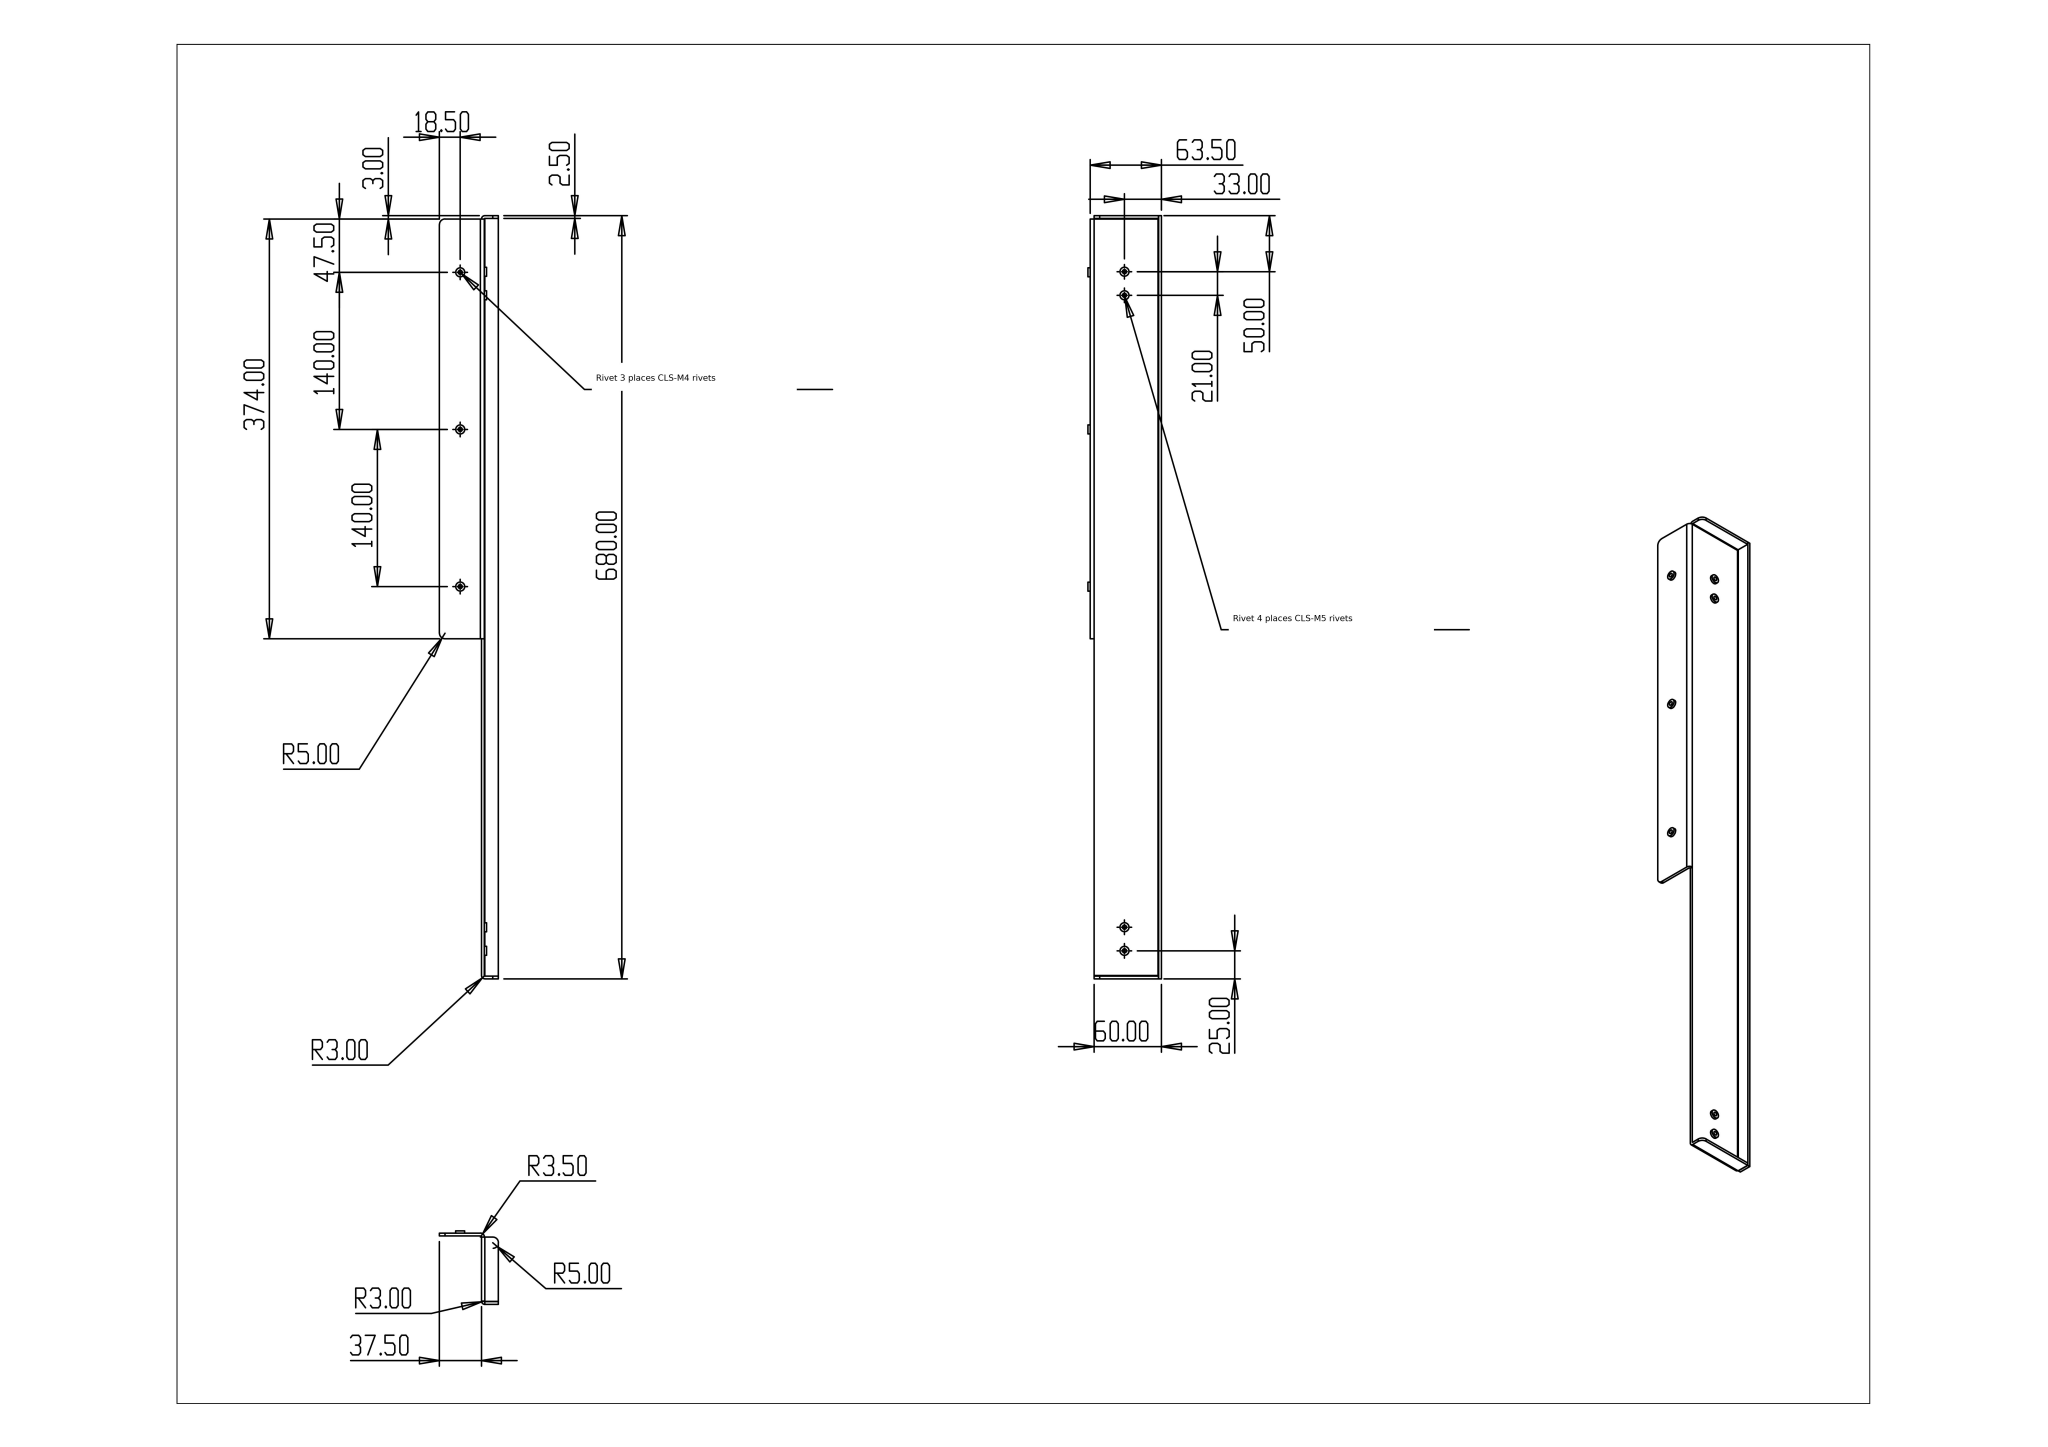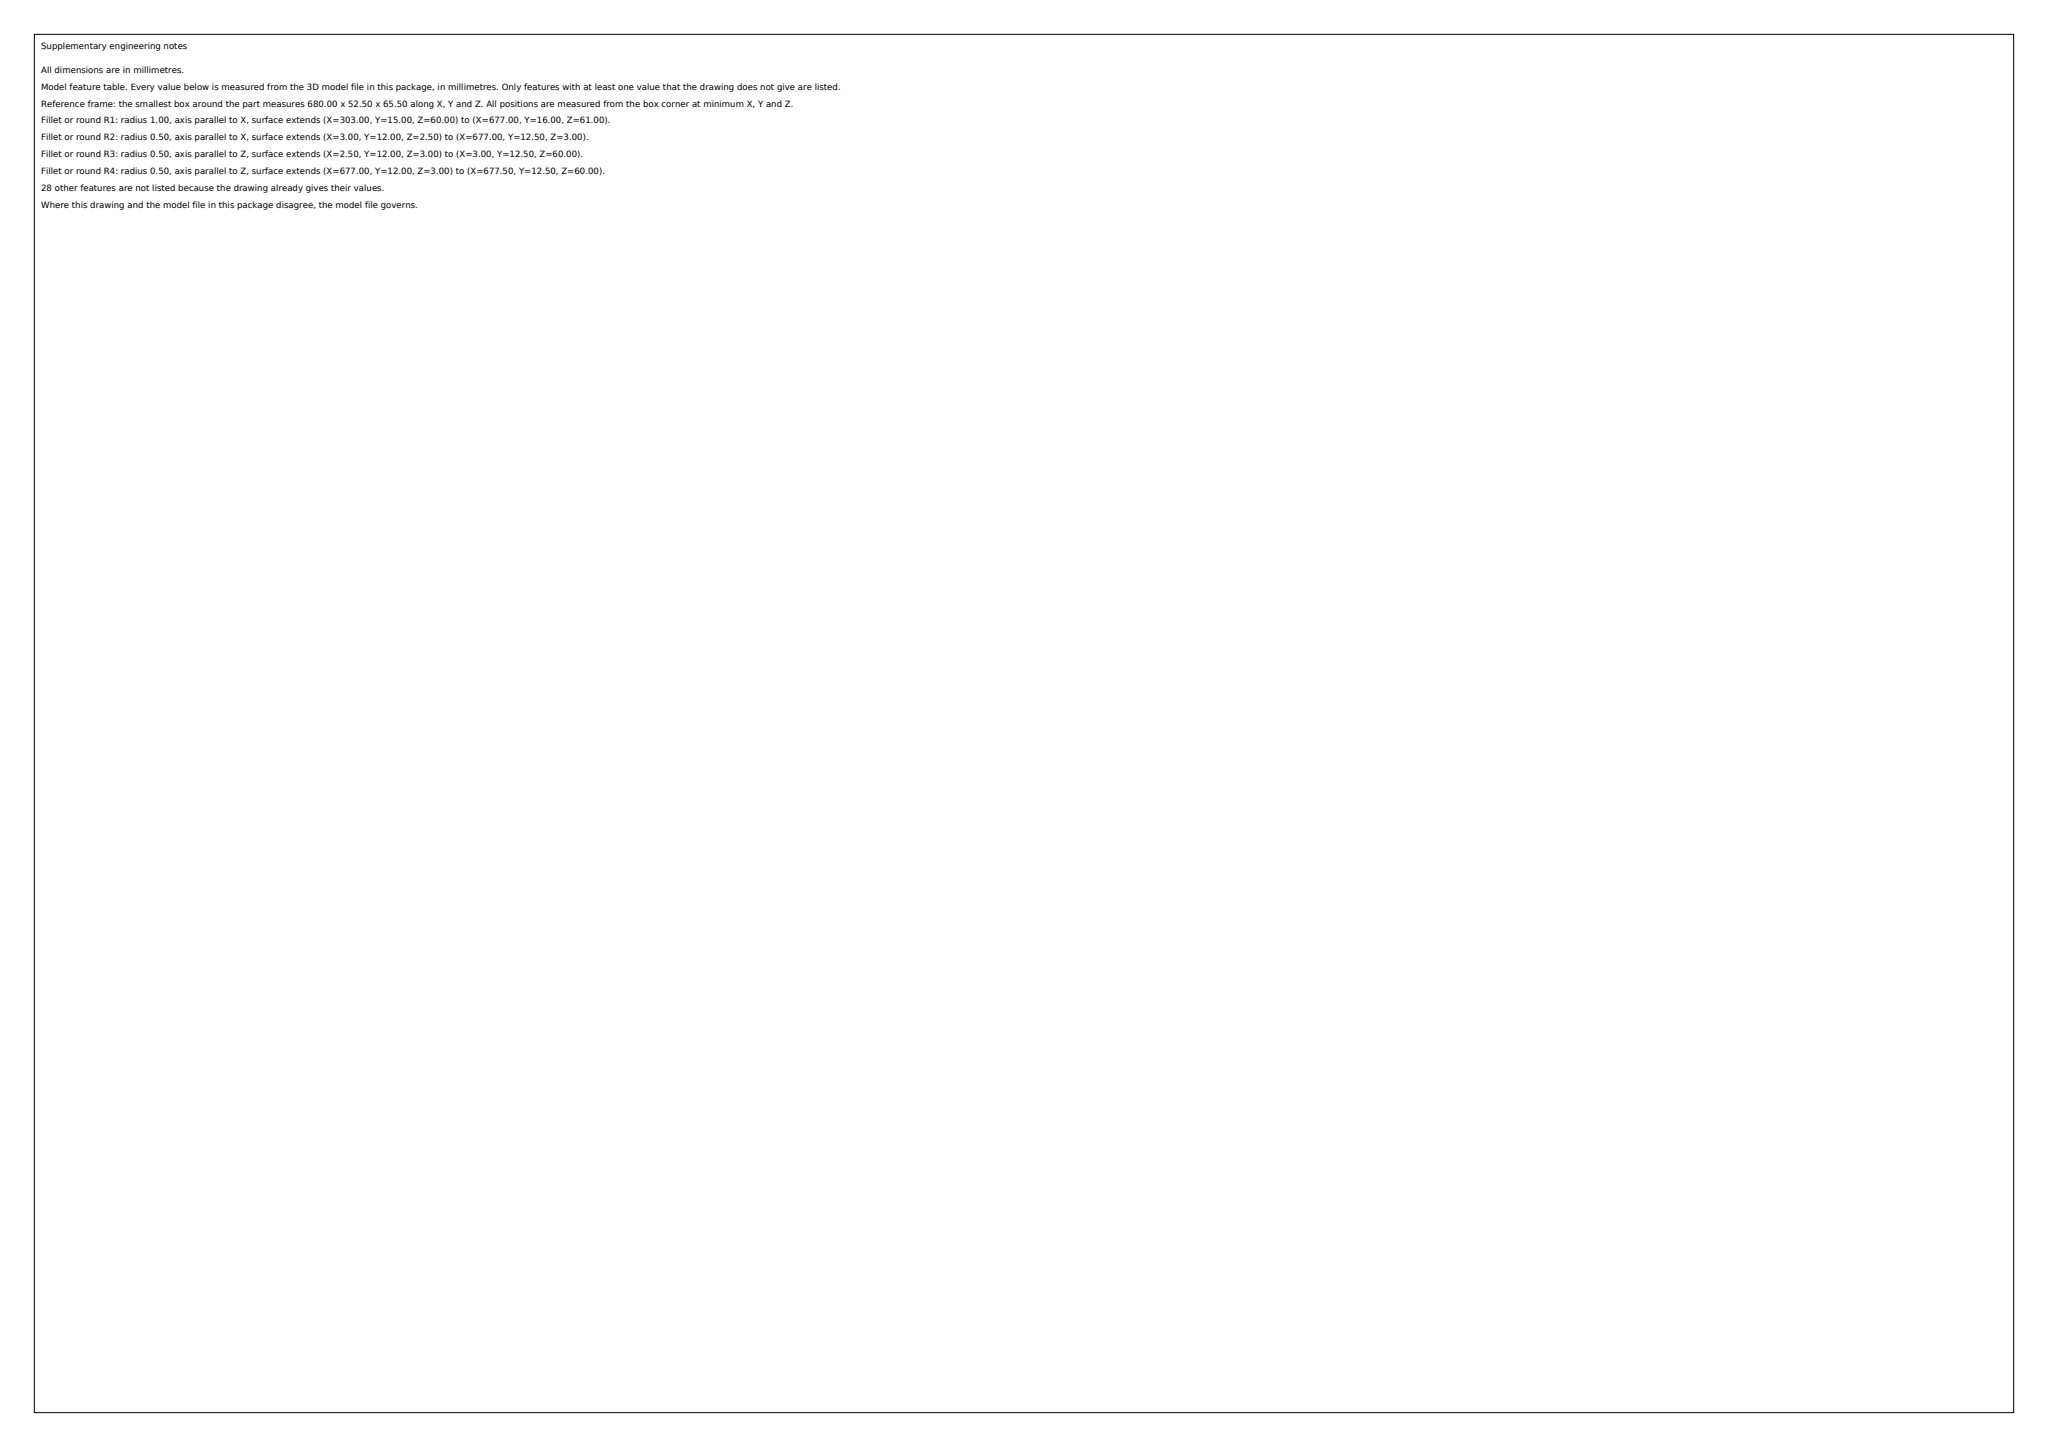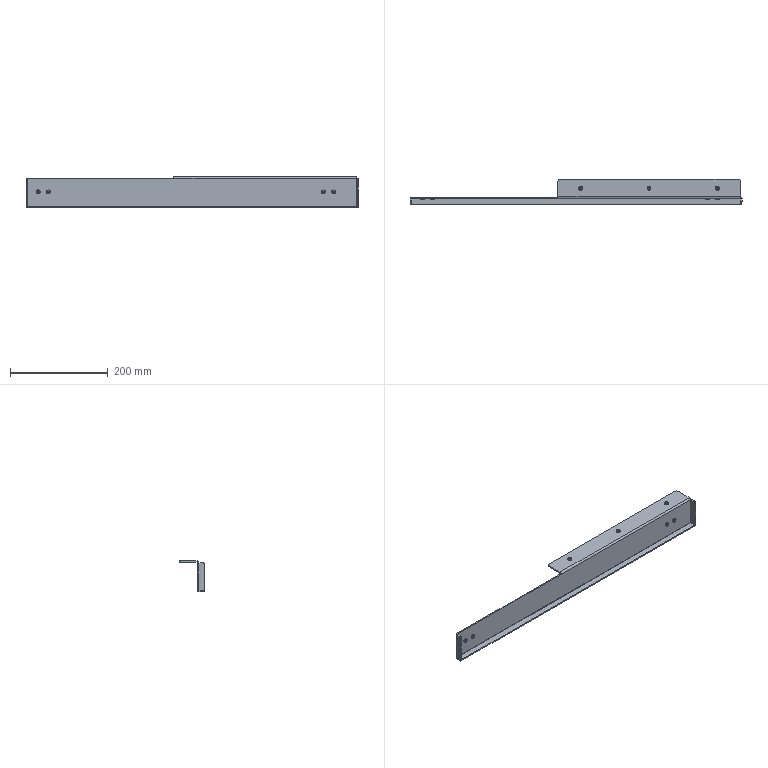Part | SolidWorks | mm | 1 solid | 98 faces | box 680 x 52.5 x 65.5 mm | volume 162932 mm3 | cylinder 54 | plane 44 | commonest cylinder face diameters 3.5 x14 8 x14 5.5 x8 5.41 x6 10 x4 6 x3 1 x3 2 x1
build123d program:
from build123d import *

# Parameters (mm, degrees)
BOSS_EXTRUDE1_DEPTH      = 57
BOSS_EXTRUDE2_DEPTH      = 374
BOSS_EXTRUDE3_DEPTH      = 674
SKETCH5_W                = 3
SKETCH5_H                = 2.5
SKETCH5_W_2              = 2.5
SKETCH5_H_2              = 0.3
BOSS_EXTRUDE4_DEPTH      = 12
FILLET1_R                = 5
CUT_EXTRUDE1_DEPTH       = 674
CUT_EXTRUDE2_DEPTH       = 674
BOSS_EXTRUDE5_DEPTH      = 2
BOSS_EXTRUDE5_DEPTH_BACK = 1
SKETCH8_R                = 4
SKETCH8_R_2              = 1.75
BOSS_EXTRUDE6_DEPTH      = 2
BOSS_EXTRUDE6_DEPTH_BACK = 1
SKETCH9_R                = 4
SKETCH9_R_2              = 1.75


with BuildPart() as part:
    # Sketch1 → Boss-Extrude1 (new body)
    with BuildSketch(Plane.XY):
        with BuildLine():
            Line((357.757, 12.959), (357.757, 7.959))
            Line((357.757, 7.959), (360.257, 7.959))
            Line((360.257, 7.959), (360.257, 12.959))
            Line((360.257, 12.959), (360.257, 19.959))
            ThreePointArc((360.257, 19.959), (359.378, 22.08), (357.257, 22.959))
            Line((357.257, 22.959), (57.257, 22.959))
            Line((57.257, 22.959), (-316.743, 22.959))
            ThreePointArc((-316.743, 22.959), (-318.864, 22.08), (-319.743, 19.959))
            Line((-319.743, 19.959), (-319.743, 12.959))
            Line((-319.743, 12.959), (-319.743, 7.959))
            Line((-319.743, 7.959), (-317.243, 7.959))
            Line((-317.243, 7.959), (-317.243, 12.959))
            Line((-317.243, 12.959), (-317.243, 19.959))
            ThreePointArc((-317.243, 19.959), (-317.097, 20.313), (-316.743, 20.459))
            Line((-316.743, 20.459), (57.257, 20.459))
            Line((57.257, 20.459), (357.257, 20.459))
            ThreePointArc((357.257, 20.459), (357.61, 20.313), (357.757, 19.959))
            Line((357.757, 19.959), (357.757, 12.959))
        make_face()
    extrude(amount=BOSS_EXTRUDE1_DEPTH)

    # Sketch3 → Boss-Extrude2 (add)
    with BuildSketch(Plane(origin=(357.257, 0, 0), x_dir=(0, 0, -1), z_dir=(1, 0, 0))):
        with BuildLine():
            Line((-57, 22.959), (-57, 20.459))
            ThreePointArc((-57, 20.459), (-59.475, 21.484), (-60.5, 23.959))
            Line((-60.5, 23.959), (-60.5, 55.459))
            Line((-60.5, 55.459), (-60.5, 60.459))
            Line((-60.5, 60.459), (-58, 60.459))
            Line((-58, 60.459), (-58, 55.459))
            Line((-58, 55.459), (-58, 23.959))
            ThreePointArc((-58, 23.959), (-57.707, 23.252), (-57, 22.959))
        make_face()
    extrude(amount=-BOSS_EXTRUDE2_DEPTH)

    # Sketch4 → Boss-Extrude3 (add)
    with BuildSketch(Plane(origin=(357.257, 0, 0), x_dir=(0, 0, -1), z_dir=(1, 0, 0))):
        with BuildLine():
            Line((0.5, 7.959), (0.5, 19.959))
            ThreePointArc((0.5, 19.959), (0.3536, 20.313), (0, 20.459))
            Line((0, 20.459), (0, 22.959))
            ThreePointArc((0, 22.959), (2.121, 22.08), (3, 19.959))
            Line((3, 19.959), (3, 7.959))
            Line((3, 7.959), (0.5, 7.959))
        make_face()
    extrude(amount=-BOSS_EXTRUDE3_DEPTH)

    # Sketch5 → Boss-Extrude4 (add)
    with BuildSketch(Plane.XZ.offset(-7.959)):
        with Locations((-318.243, -1.75)):
            Rectangle(SKETCH5_W, SKETCH5_H)
        with Locations((-318.493, -0.15)):
            Rectangle(SKETCH5_W_2, SKETCH5_H_2)
        with Locations((358.757, -1.75)):
            Rectangle(SKETCH5_W, SKETCH5_H)
        with Locations((359.007, -0.15)):
            Rectangle(SKETCH5_W_2, SKETCH5_H_2)
    extrude(amount=-BOSS_EXTRUDE4_DEPTH)

    # Fillet1
    fillet1_edges = [part.edges().sort_by_distance(p)[0] for p in [
        (359.007, 7.959, 57),
        (-318.493, 7.959, 57),
        (-16.743, 60.459, 59.25),
        (357.257, 60.459, 59.25),
    ]]
    fillet(fillet1_edges, radius=FILLET1_R)

    # Sketch6 → Cut-Extrude1 (cut)
    with BuildSketch(Plane.XY.offset(60.5)):
        with BuildLine():
            ThreePointArc((307.052, 41.959), (309.757, 39.254), (312.462, 41.959))
            ThreePointArc((312.462, 41.959), (309.757, 44.664), (307.052, 41.959))
        make_face()
        with BuildLine():
            ThreePointArc((27.052, 41.959), (29.757, 39.254), (32.462, 41.959))
            ThreePointArc((32.462, 41.959), (29.757, 44.664), (27.052, 41.959))
        make_face()
        with BuildLine():
            ThreePointArc((167.052, 41.959), (169.757, 39.254), (172.462, 41.959))
            ThreePointArc((172.462, 41.959), (169.757, 44.664), (167.052, 41.959))
        make_face()
    extrude(amount=-CUT_EXTRUDE1_DEPTH, mode=Mode.SUBTRACT)

    # Sketch7 → Cut-Extrude2 (cut)
    with BuildSketch(Plane.XZ.offset(-20.459)):
        with BuildLine():
            ThreePointArc((-276.493, 30), (-273.743, 27.25), (-270.993, 30))
            ThreePointArc((-270.993, 30), (-273.743, 32.75), (-276.493, 30))
        make_face()
        with BuildLine():
            ThreePointArc((286.507, 30), (289.257, 27.25), (292.007, 30))
            ThreePointArc((292.007, 30), (289.257, 32.75), (286.507, 30))
        make_face()
        with BuildLine():
            ThreePointArc((307.507, 30), (310.257, 27.25), (313.007, 30))
            ThreePointArc((313.007, 30), (310.257, 32.75), (307.507, 30))
        make_face()
        with BuildLine():
            ThreePointArc((-297.493, 30), (-294.743, 27.25), (-291.993, 30))
            ThreePointArc((-291.993, 30), (-294.743, 32.75), (-297.493, 30))
        make_face()
    extrude(amount=-CUT_EXTRUDE2_DEPTH, mode=Mode.SUBTRACT)

    # Sketch8 → Boss-Extrude5 (add, two sides: drawn at the far end of the back side and taken through both)
    # profile 1 of 4: a face of its own
    with BuildSketch(Plane(origin=(0, 20.459, 0), x_dir=(-1, 0, 0), z_dir=(0, -1, 0)).offset(-BOSS_EXTRUDE5_DEPTH_BACK)):
        with Locations(Location((-289.257, -30, 0), (0, 0, 180))):
            Circle(SKETCH8_R)
        with Locations(Location((-289.257, -30, 0), (0, 0, 180))):
            Circle(SKETCH8_R_2, mode=Mode.SUBTRACT)
    # profile 2 of 4: a face of its own
    with BuildSketch(Plane(origin=(0, 20.459, 0), x_dir=(-1, 0, 0), z_dir=(0, -1, 0)).offset(-BOSS_EXTRUDE5_DEPTH_BACK)):
        with Locations(Location((-310.257, -30, 0), (0, 0, 180))):
            Circle(SKETCH8_R)
        with Locations(Location((-310.257, -30, 0), (0, 0, 180))):
            Circle(SKETCH8_R_2, mode=Mode.SUBTRACT)
    # profile 3 of 4: a face of its own
    with BuildSketch(Plane(origin=(0, 20.459, 0), x_dir=(-1, 0, 0), z_dir=(0, -1, 0)).offset(-BOSS_EXTRUDE5_DEPTH_BACK)):
        with Locations(Location((294.743, -30, 0), (0, 0, 180))):
            Circle(SKETCH8_R)
        with Locations(Location((294.743, -30, 0), (0, 0, 180))):
            Circle(SKETCH8_R_2, mode=Mode.SUBTRACT)
    # profile 4 of 4: a face of its own
    with BuildSketch(Plane(origin=(0, 20.459, 0), x_dir=(-1, 0, 0), z_dir=(0, -1, 0)).offset(-BOSS_EXTRUDE5_DEPTH_BACK)):
        with Locations(Location((273.743, -30, 0), (0, 0, 180))):
            Circle(SKETCH8_R)
        with Locations(Location((273.743, -30, 0), (0, 0, 180))):
            Circle(SKETCH8_R_2, mode=Mode.SUBTRACT)
    extrude(amount=BOSS_EXTRUDE5_DEPTH + BOSS_EXTRUDE5_DEPTH_BACK)

    # Sketch9 → Boss-Extrude6 (add, two sides: drawn at the far end of the back side and taken through both)
    # profile 1 of 3: a face of its own
    with BuildSketch(Plane.XY.offset(60.5).offset(-BOSS_EXTRUDE6_DEPTH_BACK)):
        with Locations((309.757, 41.959)):
            Circle(SKETCH9_R)
        with Locations((309.757, 41.959)):
            Circle(SKETCH9_R_2, mode=Mode.SUBTRACT)
    # profile 2 of 3: a face of its own
    with BuildSketch(Plane.XY.offset(60.5).offset(-BOSS_EXTRUDE6_DEPTH_BACK)):
        with Locations((169.757, 41.959)):
            Circle(SKETCH9_R)
        with Locations((169.757, 41.959)):
            Circle(SKETCH9_R_2, mode=Mode.SUBTRACT)
    # profile 3 of 3: a face of its own
    with BuildSketch(Plane.XY.offset(60.5).offset(-BOSS_EXTRUDE6_DEPTH_BACK)):
        with Locations((29.757, 41.959)):
            Circle(SKETCH9_R)
        with Locations((29.757, 41.959)):
            Circle(SKETCH9_R_2, mode=Mode.SUBTRACT)
    extrude(amount=BOSS_EXTRUDE6_DEPTH + BOSS_EXTRUDE6_DEPTH_BACK)


solid = part.part